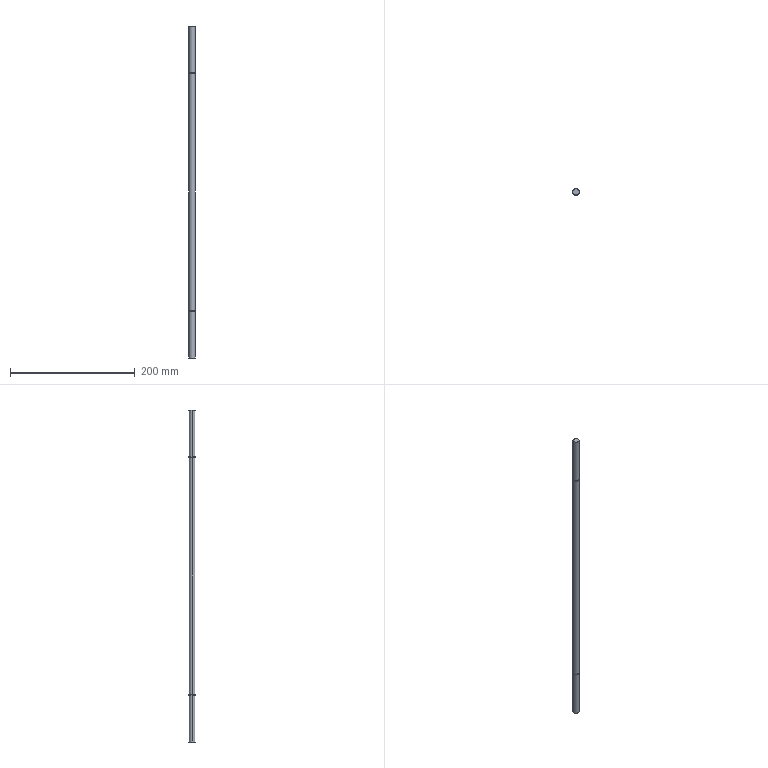Component | SolidWorks | RollerAxis3-1 | 1 solid | 16 faces | box 10 x 10 x 533 mm | volume 41850 mm3 | cylinder 10 | plane 6 | commonest cylinder face diameters 10 x6 9.65 x4
build123d program:
from build123d import *


with BuildPart() as part:
    # Sketch1 → Revolve1 (revolve)
    with BuildSketch(Plane(origin=(0, 0, 0), x_dir=(-1, 0, 0), z_dir=(0, 0, -1)), mode=Mode.PRIVATE) as revolve1_sk:
        Polygon((-266.5, 5), (-266.5, 0), (266.5, 0), (266.5, 5), (191.1, 5), (191.1, 4.825), (190, 4.825), (190, 5), (-190, 5), (-190, 4.825), (-191.1, 4.825), (-191.1, 5), align=None)
    revolve(revolve1_sk.sketch.rotate(Axis((266.5, 0, 0), (-1, 0, 0)), 270), axis=Axis((266.5, 0, 0), (-1, 0, 0)))


solid = part.part

# Placed as in the assembly
solid = solid.moved(Location((318, 551, 0), (0, 90, 0)))
STEP:
#1=COLOUR_RGB('',0.7922,0.8196,0.9333);
#2=FILL_AREA_STYLE_COLOUR('',#1);
#3=FILL_AREA_STYLE('',(#2));
#4=SURFACE_STYLE_FILL_AREA(#3);
#5=SURFACE_SIDE_STYLE('',(#4));
#6=SURFACE_STYLE_USAGE(.BOTH.,#5);
#7=PRESENTATION_STYLE_ASSIGNMENT((#6));
#8=CARTESIAN_POINT('',(12.33,21.693,7.524));
#9=VERTEX_POINT('',#8);
#10=CARTESIAN_POINT('',(12.71,21.693,7.524));
#11=VERTEX_POINT('',#10);
#12=CARTESIAN_POINT('',(12.52,21.693,7.524));
#13=DIRECTION('',(-0.,0.,-1.));
#14=DIRECTION('',(-1.,0.,0.));
#15=AXIS2_PLACEMENT_3D('',#12,#13,#14);
#16=CIRCLE('',#15,0.19);
#17=EDGE_CURVE('',#9,#11,#16,.T.);
#18=ORIENTED_EDGE('',*,*,#17,.T.);
#19=CARTESIAN_POINT('',(12.71,21.693,7.48));
#20=VERTEX_POINT('',#19);
#21=CARTESIAN_POINT('',(12.71,21.693,10.492));
#22=DIRECTION('',(-0.,0.,-1.));
#23=VECTOR('',#22,39.37);
#24=LINE('',#21,#23);
#25=EDGE_CURVE('',#11,#20,#24,.T.);
#26=ORIENTED_EDGE('',*,*,#25,.T.);
#27=CARTESIAN_POINT('',(12.33,21.693,7.48));
#28=VERTEX_POINT('',#27);
#29=CARTESIAN_POINT('',(12.52,21.693,7.48));
#30=DIRECTION('',(-0.,0.,-1.));
#31=DIRECTION('',(-1.,0.,0.));
#32=AXIS2_PLACEMENT_3D('',#29,#30,#31);
#33=CIRCLE('',#32,0.19);
#34=EDGE_CURVE('',#28,#20,#33,.T.);
#35=ORIENTED_EDGE('',*,*,#34,.F.);
#36=CARTESIAN_POINT('',(12.33,21.693,10.492));
#37=DIRECTION('',(-0.,0.,-1.));
#38=VECTOR('',#37,39.37);
#39=LINE('',#36,#38);
#40=EDGE_CURVE('',#9,#28,#39,.T.);
#41=ORIENTED_EDGE('',*,*,#40,.F.);
#42=EDGE_LOOP('',(#18,#26,#35,#41));
#43=FACE_OUTER_BOUND('',#42,.T.);
#44=CARTESIAN_POINT('',(12.52,21.693,10.492));
#45=DIRECTION('',(-0.,0.,-1.));
#46=DIRECTION('',(-1.,0.,0.));
#47=AXIS2_PLACEMENT_3D('',#44,#45,#46);
#48=CYLINDRICAL_SURFACE('',#47,0.19);
#49=ADVANCED_FACE('',(#43),#48,.T.);
#50=CARTESIAN_POINT('',(12.323,21.693,7.48));
#51=VERTEX_POINT('',#50);
#52=CARTESIAN_POINT('',(12.717,21.693,7.48));
#53=VERTEX_POINT('',#52);
#54=CARTESIAN_POINT('',(12.52,21.693,7.48));
#55=DIRECTION('',(-0.,0.,-1.));
#56=DIRECTION('',(-1.,0.,0.));
#57=AXIS2_PLACEMENT_3D('',#54,#55,#56);
#58=CIRCLE('',#57,0.1969);
#59=EDGE_CURVE('',#51,#53,#58,.T.);
#60=ORIENTED_EDGE('',*,*,#59,.T.);
#61=CARTESIAN_POINT('',(12.717,21.693,-7.48));
#62=VERTEX_POINT('',#61);
#63=CARTESIAN_POINT('',(12.717,21.693,10.492));
#64=DIRECTION('',(-0.,0.,-1.));
#65=VECTOR('',#64,39.37);
#66=LINE('',#63,#65);
#67=EDGE_CURVE('',#53,#62,#66,.T.);
#68=ORIENTED_EDGE('',*,*,#67,.T.);
#69=CARTESIAN_POINT('',(12.323,21.693,-7.48));
#70=VERTEX_POINT('',#69);
#71=CARTESIAN_POINT('',(12.52,21.693,-7.48));
#72=DIRECTION('',(-0.,0.,-1.));
#73=DIRECTION('',(-1.,0.,0.));
#74=AXIS2_PLACEMENT_3D('',#71,#72,#73);
#75=CIRCLE('',#74,0.1969);
#76=EDGE_CURVE('',#70,#62,#75,.T.);
#77=ORIENTED_EDGE('',*,*,#76,.F.);
#78=CARTESIAN_POINT('',(12.323,21.693,10.492));
#79=DIRECTION('',(-0.,0.,-1.));
#80=VECTOR('',#79,39.37);
#81=LINE('',#78,#80);
#82=EDGE_CURVE('',#51,#70,#81,.T.);
#83=ORIENTED_EDGE('',*,*,#82,.F.);
#84=EDGE_LOOP('',(#60,#68,#77,#83));
#85=FACE_OUTER_BOUND('',#84,.T.);
#86=CARTESIAN_POINT('',(12.52,21.693,10.492));
#87=DIRECTION('',(-0.,0.,-1.));
#88=DIRECTION('',(-1.,0.,0.));
#89=AXIS2_PLACEMENT_3D('',#86,#87,#88);
#90=CYLINDRICAL_SURFACE('',#89,0.1969);
#91=ADVANCED_FACE('',(#85),#90,.T.);
#92=CARTESIAN_POINT('',(12.33,21.693,-7.48));
#93=VERTEX_POINT('',#92);
#94=CARTESIAN_POINT('',(12.71,21.693,-7.48));
#95=VERTEX_POINT('',#94);
#96=CARTESIAN_POINT('',(12.52,21.693,-7.48));
#97=DIRECTION('',(-0.,0.,-1.));
#98=DIRECTION('',(-1.,0.,0.));
#99=AXIS2_PLACEMENT_3D('',#96,#97,#98);
#100=CIRCLE('',#99,0.19);
#101=EDGE_CURVE('',#93,#95,#100,.T.);
#102=ORIENTED_EDGE('',*,*,#101,.T.);
#103=CARTESIAN_POINT('',(12.71,21.693,-7.524));
#104=VERTEX_POINT('',#103);
#105=CARTESIAN_POINT('',(12.71,21.693,10.492));
#106=DIRECTION('',(-0.,0.,-1.));
#107=VECTOR('',#106,39.37);
#108=LINE('',#105,#107);
#109=EDGE_CURVE('',#95,#104,#108,.T.);
#110=ORIENTED_EDGE('',*,*,#109,.T.);
#111=CARTESIAN_POINT('',(12.33,21.693,-7.524));
#112=VERTEX_POINT('',#111);
#113=CARTESIAN_POINT('',(12.52,21.693,-7.524));
#114=DIRECTION('',(-0.,0.,-1.));
#115=DIRECTION('',(-1.,0.,0.));
#116=AXIS2_PLACEMENT_3D('',#113,#114,#115);
#117=CIRCLE('',#116,0.19);
#118=EDGE_CURVE('',#112,#104,#117,.T.);
#119=ORIENTED_EDGE('',*,*,#118,.F.);
#120=CARTESIAN_POINT('',(12.33,21.693,10.492));
#121=DIRECTION('',(-0.,0.,-1.));
#122=VECTOR('',#121,39.37);
#123=LINE('',#120,#122);
#124=EDGE_CURVE('',#93,#112,#123,.T.);
#125=ORIENTED_EDGE('',*,*,#124,.F.);
#126=EDGE_LOOP('',(#102,#110,#119,#125));
#127=FACE_OUTER_BOUND('',#126,.T.);
#128=CARTESIAN_POINT('',(12.52,21.693,10.492));
#129=DIRECTION('',(-0.,0.,-1.));
#130=DIRECTION('',(-1.,0.,0.));
#131=AXIS2_PLACEMENT_3D('',#128,#129,#130);
#132=CYLINDRICAL_SURFACE('',#131,0.19);
#133=ADVANCED_FACE('',(#127),#132,.T.);
#134=CARTESIAN_POINT('',(12.323,21.693,-7.524));
#135=VERTEX_POINT('',#134);
#136=CARTESIAN_POINT('',(12.717,21.693,-7.524));
#137=VERTEX_POINT('',#136);
#138=CARTESIAN_POINT('',(12.52,21.693,-7.524));
#139=DIRECTION('',(-0.,0.,-1.));
#140=DIRECTION('',(-1.,0.,0.));
#141=AXIS2_PLACEMENT_3D('',#138,#139,#140);
#142=CIRCLE('',#141,0.1969);
#143=EDGE_CURVE('',#135,#137,#142,.T.);
#144=ORIENTED_EDGE('',*,*,#143,.T.);
#145=CARTESIAN_POINT('',(12.717,21.693,-10.492));
#146=VERTEX_POINT('',#145);
#147=CARTESIAN_POINT('',(12.717,21.693,10.492));
#148=DIRECTION('',(-0.,0.,-1.));
#149=VECTOR('',#148,39.37);
#150=LINE('',#147,#149);
#151=EDGE_CURVE('',#137,#146,#150,.T.);
#152=ORIENTED_EDGE('',*,*,#151,.T.);
#153=CARTESIAN_POINT('',(12.323,21.693,-10.492));
#154=VERTEX_POINT('',#153);
#155=CARTESIAN_POINT('',(12.52,21.693,-10.492));
#156=DIRECTION('',(-0.,0.,-1.));
#157=DIRECTION('',(-1.,0.,0.));
#158=AXIS2_PLACEMENT_3D('',#155,#156,#157);
#159=CIRCLE('',#158,0.1969);
#160=EDGE_CURVE('',#154,#146,#159,.T.);
#161=ORIENTED_EDGE('',*,*,#160,.F.);
#162=CARTESIAN_POINT('',(12.323,21.693,10.492));
#163=DIRECTION('',(-0.,0.,-1.));
#164=VECTOR('',#163,39.37);
#165=LINE('',#162,#164);
#166=EDGE_CURVE('',#135,#154,#165,.T.);
#167=ORIENTED_EDGE('',*,*,#166,.F.);
#168=EDGE_LOOP('',(#144,#152,#161,#167));
#169=FACE_OUTER_BOUND('',#168,.T.);
#170=CARTESIAN_POINT('',(12.52,21.693,10.492));
#171=DIRECTION('',(-0.,0.,-1.));
#172=DIRECTION('',(-1.,0.,0.));
#173=AXIS2_PLACEMENT_3D('',#170,#171,#172);
#174=CYLINDRICAL_SURFACE('',#173,0.1969);
#175=ADVANCED_FACE('',(#169),#174,.T.);
#176=CARTESIAN_POINT('',(12.323,21.693,10.492));
#177=VERTEX_POINT('',#176);
#178=CARTESIAN_POINT('',(12.717,21.693,10.492));
#179=VERTEX_POINT('',#178);
#180=CARTESIAN_POINT('',(12.52,21.693,10.492));
#181=DIRECTION('',(-0.,0.,-1.));
#182=DIRECTION('',(-1.,0.,0.));
#183=AXIS2_PLACEMENT_3D('',#180,#181,#182);
#184=CIRCLE('',#183,0.1969);
#185=EDGE_CURVE('',#177,#179,#184,.T.);
#186=ORIENTED_EDGE('',*,*,#185,.T.);
#187=CARTESIAN_POINT('',(12.717,21.693,7.524));
#188=VERTEX_POINT('',#187);
#189=CARTESIAN_POINT('',(12.717,21.693,10.492));
#190=DIRECTION('',(-0.,0.,-1.));
#191=VECTOR('',#190,39.37);
#192=LINE('',#189,#191);
#193=EDGE_CURVE('',#179,#188,#192,.T.);
#194=ORIENTED_EDGE('',*,*,#193,.T.);
#195=CARTESIAN_POINT('',(12.323,21.693,7.524));
#196=VERTEX_POINT('',#195);
#197=CARTESIAN_POINT('',(12.52,21.693,7.524));
#198=DIRECTION('',(-0.,0.,-1.));
#199=DIRECTION('',(-1.,0.,0.));
#200=AXIS2_PLACEMENT_3D('',#197,#198,#199);
#201=CIRCLE('',#200,0.1969);
#202=EDGE_CURVE('',#196,#188,#201,.T.);
#203=ORIENTED_EDGE('',*,*,#202,.F.);
#204=CARTESIAN_POINT('',(12.323,21.693,10.492));
#205=DIRECTION('',(-0.,0.,-1.));
#206=VECTOR('',#205,39.37);
#207=LINE('',#204,#206);
#208=EDGE_CURVE('',#177,#196,#207,.T.);
#209=ORIENTED_EDGE('',*,*,#208,.F.);
#210=EDGE_LOOP('',(#186,#194,#203,#209));
#211=FACE_OUTER_BOUND('',#210,.T.);
#212=CARTESIAN_POINT('',(12.52,21.693,10.492));
#213=DIRECTION('',(-0.,0.,-1.));
#214=DIRECTION('',(-1.,0.,0.));
#215=AXIS2_PLACEMENT_3D('',#212,#213,#214);
#216=CYLINDRICAL_SURFACE('',#215,0.1969);
#217=ADVANCED_FACE('',(#211),#216,.T.);
#218=ORIENTED_EDGE('',*,*,#193,.F.);
#219=CARTESIAN_POINT('',(12.52,21.693,10.492));
#220=DIRECTION('',(-0.,0.,-1.));
#221=DIRECTION('',(-1.,0.,0.));
#222=AXIS2_PLACEMENT_3D('',#219,#220,#221);
#223=CIRCLE('',#222,0.1969);
#224=EDGE_CURVE('',#179,#177,#223,.T.);
#225=ORIENTED_EDGE('',*,*,#224,.T.);
#226=ORIENTED_EDGE('',*,*,#208,.T.);
#227=CARTESIAN_POINT('',(12.52,21.693,7.524));
#228=DIRECTION('',(-0.,0.,-1.));
#229=DIRECTION('',(-1.,0.,0.));
#230=AXIS2_PLACEMENT_3D('',#227,#228,#229);
#231=CIRCLE('',#230,0.1969);
#232=EDGE_CURVE('',#188,#196,#231,.T.);
#233=ORIENTED_EDGE('',*,*,#232,.F.);
#234=EDGE_LOOP('',(#218,#225,#226,#233));
#235=FACE_OUTER_BOUND('',#234,.T.);
#236=CARTESIAN_POINT('',(12.52,21.693,10.492));
#237=DIRECTION('',(-0.,0.,-1.));
#238=DIRECTION('',(-1.,0.,0.));
#239=AXIS2_PLACEMENT_3D('',#236,#237,#238);
#240=CYLINDRICAL_SURFACE('',#239,0.1969);
#241=ADVANCED_FACE('',(#235),#240,.T.);
#242=ORIENTED_EDGE('',*,*,#185,.F.);
#243=ORIENTED_EDGE('',*,*,#224,.F.);
#244=EDGE_LOOP('',(#242,#243));
#245=FACE_OUTER_BOUND('',#244,.T.);
#246=CARTESIAN_POINT('',(12.52,21.89,10.492));
#247=DIRECTION('',(0.,0.,1.));
#248=DIRECTION('',(1.,0.,-0.));
#249=AXIS2_PLACEMENT_3D('',#246,#247,#248);
#250=PLANE('',#249);
#251=ADVANCED_FACE('',(#245),#250,.T.);
#252=ORIENTED_EDGE('',*,*,#160,.T.);
#253=CARTESIAN_POINT('',(12.52,21.693,-10.492));
#254=DIRECTION('',(-0.,0.,-1.));
#255=DIRECTION('',(-1.,0.,0.));
#256=AXIS2_PLACEMENT_3D('',#253,#254,#255);
#257=CIRCLE('',#256,0.1969);
#258=EDGE_CURVE('',#146,#154,#257,.T.);
#259=ORIENTED_EDGE('',*,*,#258,.T.);
#260=EDGE_LOOP('',(#252,#259));
#261=FACE_OUTER_BOUND('',#260,.T.);
#262=CARTESIAN_POINT('',(12.52,21.693,-10.492));
#263=DIRECTION('',(-0.,0.,-1.));
#264=DIRECTION('',(-1.,0.,0.));
#265=AXIS2_PLACEMENT_3D('',#262,#263,#264);
#266=PLANE('',#265);
#267=ADVANCED_FACE('',(#261),#266,.T.);
#268=ORIENTED_EDGE('',*,*,#151,.F.);
#269=CARTESIAN_POINT('',(12.52,21.693,-7.524));
#270=DIRECTION('',(-0.,0.,-1.));
#271=DIRECTION('',(-1.,0.,0.));
#272=AXIS2_PLACEMENT_3D('',#269,#270,#271);
#273=CIRCLE('',#272,0.1969);
#274=EDGE_CURVE('',#137,#135,#273,.T.);
#275=ORIENTED_EDGE('',*,*,#274,.T.);
#276=ORIENTED_EDGE('',*,*,#166,.T.);
#277=ORIENTED_EDGE('',*,*,#258,.F.);
#278=EDGE_LOOP('',(#268,#275,#276,#277));
#279=FACE_OUTER_BOUND('',#278,.T.);
#280=CARTESIAN_POINT('',(12.52,21.693,10.492));
#281=DIRECTION('',(-0.,0.,-1.));
#282=DIRECTION('',(-1.,0.,0.));
#283=AXIS2_PLACEMENT_3D('',#280,#281,#282);
#284=CYLINDRICAL_SURFACE('',#283,0.1969);
#285=ADVANCED_FACE('',(#279),#284,.T.);
#286=ORIENTED_EDGE('',*,*,#118,.T.);
#287=CARTESIAN_POINT('',(12.52,21.693,-7.524));
#288=DIRECTION('',(-0.,0.,-1.));
#289=DIRECTION('',(-1.,0.,0.));
#290=AXIS2_PLACEMENT_3D('',#287,#288,#289);
#291=CIRCLE('',#290,0.19);
#292=EDGE_CURVE('',#104,#112,#291,.T.);
#293=ORIENTED_EDGE('',*,*,#292,.T.);
#294=EDGE_LOOP('',(#286,#293));
#295=FACE_BOUND('',#294,.T.);
#296=ORIENTED_EDGE('',*,*,#143,.F.);
#297=ORIENTED_EDGE('',*,*,#274,.F.);
#298=EDGE_LOOP('',(#296,#297));
#299=FACE_OUTER_BOUND('',#298,.T.);
#300=CARTESIAN_POINT('',(12.52,21.89,-7.524));
#301=DIRECTION('',(0.,0.,1.));
#302=DIRECTION('',(1.,0.,-0.));
#303=AXIS2_PLACEMENT_3D('',#300,#301,#302);
#304=PLANE('',#303);
#305=ADVANCED_FACE('',(#295,#299),#304,.T.);
#306=ORIENTED_EDGE('',*,*,#109,.F.);
#307=CARTESIAN_POINT('',(12.52,21.693,-7.48));
#308=DIRECTION('',(-0.,0.,-1.));
#309=DIRECTION('',(-1.,0.,0.));
#310=AXIS2_PLACEMENT_3D('',#307,#308,#309);
#311=CIRCLE('',#310,0.19);
#312=EDGE_CURVE('',#95,#93,#311,.T.);
#313=ORIENTED_EDGE('',*,*,#312,.T.);
#314=ORIENTED_EDGE('',*,*,#124,.T.);
#315=ORIENTED_EDGE('',*,*,#292,.F.);
#316=EDGE_LOOP('',(#306,#313,#314,#315));
#317=FACE_OUTER_BOUND('',#316,.T.);
#318=CARTESIAN_POINT('',(12.52,21.693,10.492));
#319=DIRECTION('',(-0.,0.,-1.));
#320=DIRECTION('',(-1.,0.,0.));
#321=AXIS2_PLACEMENT_3D('',#318,#319,#320);
#322=CYLINDRICAL_SURFACE('',#321,0.19);
#323=ADVANCED_FACE('',(#317),#322,.T.);
#324=ORIENTED_EDGE('',*,*,#76,.T.);
#325=CARTESIAN_POINT('',(12.52,21.693,-7.48));
#326=DIRECTION('',(-0.,0.,-1.));
#327=DIRECTION('',(-1.,0.,0.));
#328=AXIS2_PLACEMENT_3D('',#325,#326,#327);
#329=CIRCLE('',#328,0.1969);
#330=EDGE_CURVE('',#62,#70,#329,.T.);
#331=ORIENTED_EDGE('',*,*,#330,.T.);
#332=EDGE_LOOP('',(#324,#331));
#333=FACE_OUTER_BOUND('',#332,.T.);
#334=ORIENTED_EDGE('',*,*,#101,.F.);
#335=ORIENTED_EDGE('',*,*,#312,.F.);
#336=EDGE_LOOP('',(#334,#335));
#337=FACE_BOUND('',#336,.T.);
#338=CARTESIAN_POINT('',(12.52,21.883,-7.48));
#339=DIRECTION('',(-0.,0.,-1.));
#340=DIRECTION('',(-1.,0.,0.));
#341=AXIS2_PLACEMENT_3D('',#338,#339,#340);
#342=PLANE('',#341);
#343=ADVANCED_FACE('',(#333,#337),#342,.T.);
#344=ORIENTED_EDGE('',*,*,#67,.F.);
#345=CARTESIAN_POINT('',(12.52,21.693,7.48));
#346=DIRECTION('',(-0.,0.,-1.));
#347=DIRECTION('',(-1.,0.,0.));
#348=AXIS2_PLACEMENT_3D('',#345,#346,#347);
#349=CIRCLE('',#348,0.1969);
#350=EDGE_CURVE('',#53,#51,#349,.T.);
#351=ORIENTED_EDGE('',*,*,#350,.T.);
#352=ORIENTED_EDGE('',*,*,#82,.T.);
#353=ORIENTED_EDGE('',*,*,#330,.F.);
#354=EDGE_LOOP('',(#344,#351,#352,#353));
#355=FACE_OUTER_BOUND('',#354,.T.);
#356=CARTESIAN_POINT('',(12.52,21.693,10.492));
#357=DIRECTION('',(-0.,0.,-1.));
#358=DIRECTION('',(-1.,0.,0.));
#359=AXIS2_PLACEMENT_3D('',#356,#357,#358);
#360=CYLINDRICAL_SURFACE('',#359,0.1969);
#361=ADVANCED_FACE('',(#355),#360,.T.);
#362=ORIENTED_EDGE('',*,*,#34,.T.);
#363=CARTESIAN_POINT('',(12.52,21.693,7.48));
#364=DIRECTION('',(-0.,0.,-1.));
#365=DIRECTION('',(-1.,0.,0.));
#366=AXIS2_PLACEMENT_3D('',#363,#364,#365);
#367=CIRCLE('',#366,0.19);
#368=EDGE_CURVE('',#20,#28,#367,.T.);
#369=ORIENTED_EDGE('',*,*,#368,.T.);
#370=EDGE_LOOP('',(#362,#369));
#371=FACE_BOUND('',#370,.T.);
#372=ORIENTED_EDGE('',*,*,#59,.F.);
#373=ORIENTED_EDGE('',*,*,#350,.F.);
#374=EDGE_LOOP('',(#372,#373));
#375=FACE_OUTER_BOUND('',#374,.T.);
#376=CARTESIAN_POINT('',(12.52,21.89,7.48));
#377=DIRECTION('',(0.,0.,1.));
#378=DIRECTION('',(1.,0.,-0.));
#379=AXIS2_PLACEMENT_3D('',#376,#377,#378);
#380=PLANE('',#379);
#381=ADVANCED_FACE('',(#371,#375),#380,.T.);
#382=ORIENTED_EDGE('',*,*,#25,.F.);
#383=CARTESIAN_POINT('',(12.52,21.693,7.524));
#384=DIRECTION('',(-0.,0.,-1.));
#385=DIRECTION('',(-1.,0.,0.));
#386=AXIS2_PLACEMENT_3D('',#383,#384,#385);
#387=CIRCLE('',#386,0.19);
#388=EDGE_CURVE('',#11,#9,#387,.T.);
#389=ORIENTED_EDGE('',*,*,#388,.T.);
#390=ORIENTED_EDGE('',*,*,#40,.T.);
#391=ORIENTED_EDGE('',*,*,#368,.F.);
#392=EDGE_LOOP('',(#382,#389,#390,#391));
#393=FACE_OUTER_BOUND('',#392,.T.);
#394=CARTESIAN_POINT('',(12.52,21.693,10.492));
#395=DIRECTION('',(-0.,0.,-1.));
#396=DIRECTION('',(-1.,0.,0.));
#397=AXIS2_PLACEMENT_3D('',#394,#395,#396);
#398=CYLINDRICAL_SURFACE('',#397,0.19);
#399=ADVANCED_FACE('',(#393),#398,.T.);
#400=ORIENTED_EDGE('',*,*,#202,.T.);
#401=ORIENTED_EDGE('',*,*,#232,.T.);
#402=EDGE_LOOP('',(#400,#401));
#403=FACE_OUTER_BOUND('',#402,.T.);
#404=ORIENTED_EDGE('',*,*,#17,.F.);
#405=ORIENTED_EDGE('',*,*,#388,.F.);
#406=EDGE_LOOP('',(#404,#405));
#407=FACE_BOUND('',#406,.T.);
#408=CARTESIAN_POINT('',(12.52,21.883,7.524));
#409=DIRECTION('',(-0.,0.,-1.));
#410=DIRECTION('',(-1.,0.,0.));
#411=AXIS2_PLACEMENT_3D('',#408,#409,#410);
#412=PLANE('',#411);
#413=ADVANCED_FACE('',(#403,#407),#412,.T.);
#414=CLOSED_SHELL('',(#49,#91,#133,#175,#217,#241,#251,#267,#285,#305,#323,#343,#361,#381,#399,#413));
#415=MANIFOLD_SOLID_BREP('',#414);
#416=STYLED_ITEM('',(#7),#415);
#417=(LENGTH_UNIT()NAMED_UNIT(*)SI_UNIT($,.METRE.));
#418=LENGTH_MEASURE_WITH_UNIT(LENGTH_MEASURE(0.0254),#417);
#419=DIMENSIONAL_EXPONENTS(1.,0.,0.,0.,0.,0.,0.);
#420=(CONVERSION_BASED_UNIT('',#418)LENGTH_UNIT()NAMED_UNIT(#419));
#421=UNCERTAINTY_MEASURE_WITH_UNIT(LENGTH_MEASURE(0.00001),#420,'','');
#422=(NAMED_UNIT(*)PLANE_ANGLE_UNIT()SI_UNIT($,.RADIAN.));
#423=(NAMED_UNIT(*)SI_UNIT($,.STERADIAN.)SOLID_ANGLE_UNIT());
#424=(GEOMETRIC_REPRESENTATION_CONTEXT(3)GLOBAL_UNCERTAINTY_ASSIGNED_CONTEXT((#421))GLOBAL_UNIT_ASSIGNED_CONTEXT((#420,#422,#423))REPRESENTATION_CONTEXT('',''));
#425=MECHANICAL_DESIGN_GEOMETRIC_PRESENTATION_REPRESENTATION('',(#416),#424);
#426=CARTESIAN_POINT('',(0.,0.,0.));
#427=DIRECTION('',(0.,0.,1.));
#428=DIRECTION('',(1.,0.,0.));
#429=AXIS2_PLACEMENT_3D('',#426,#427,#428);
#430=(LENGTH_UNIT()NAMED_UNIT(*)SI_UNIT($,.METRE.));
#431=LENGTH_MEASURE_WITH_UNIT(LENGTH_MEASURE(0.0254),#430);
#432=DIMENSIONAL_EXPONENTS(1.,0.,0.,0.,0.,0.,0.);
#433=(CONVERSION_BASED_UNIT('',#431)LENGTH_UNIT()NAMED_UNIT(#432));
#434=UNCERTAINTY_MEASURE_WITH_UNIT(LENGTH_MEASURE(0.00001),#433,'','');
#435=(NAMED_UNIT(*)PLANE_ANGLE_UNIT()SI_UNIT($,.RADIAN.));
#436=(NAMED_UNIT(*)SI_UNIT($,.STERADIAN.)SOLID_ANGLE_UNIT());
#437=(GEOMETRIC_REPRESENTATION_CONTEXT(3)GLOBAL_UNCERTAINTY_ASSIGNED_CONTEXT((#434))GLOBAL_UNIT_ASSIGNED_CONTEXT((#433,#435,#436))REPRESENTATION_CONTEXT('',''));
#438=ADVANCED_BREP_SHAPE_REPRESENTATION('',(#415,#429),#437);
#439=PRESENTATION_LAYER_ASSIGNMENT('','',(#416));